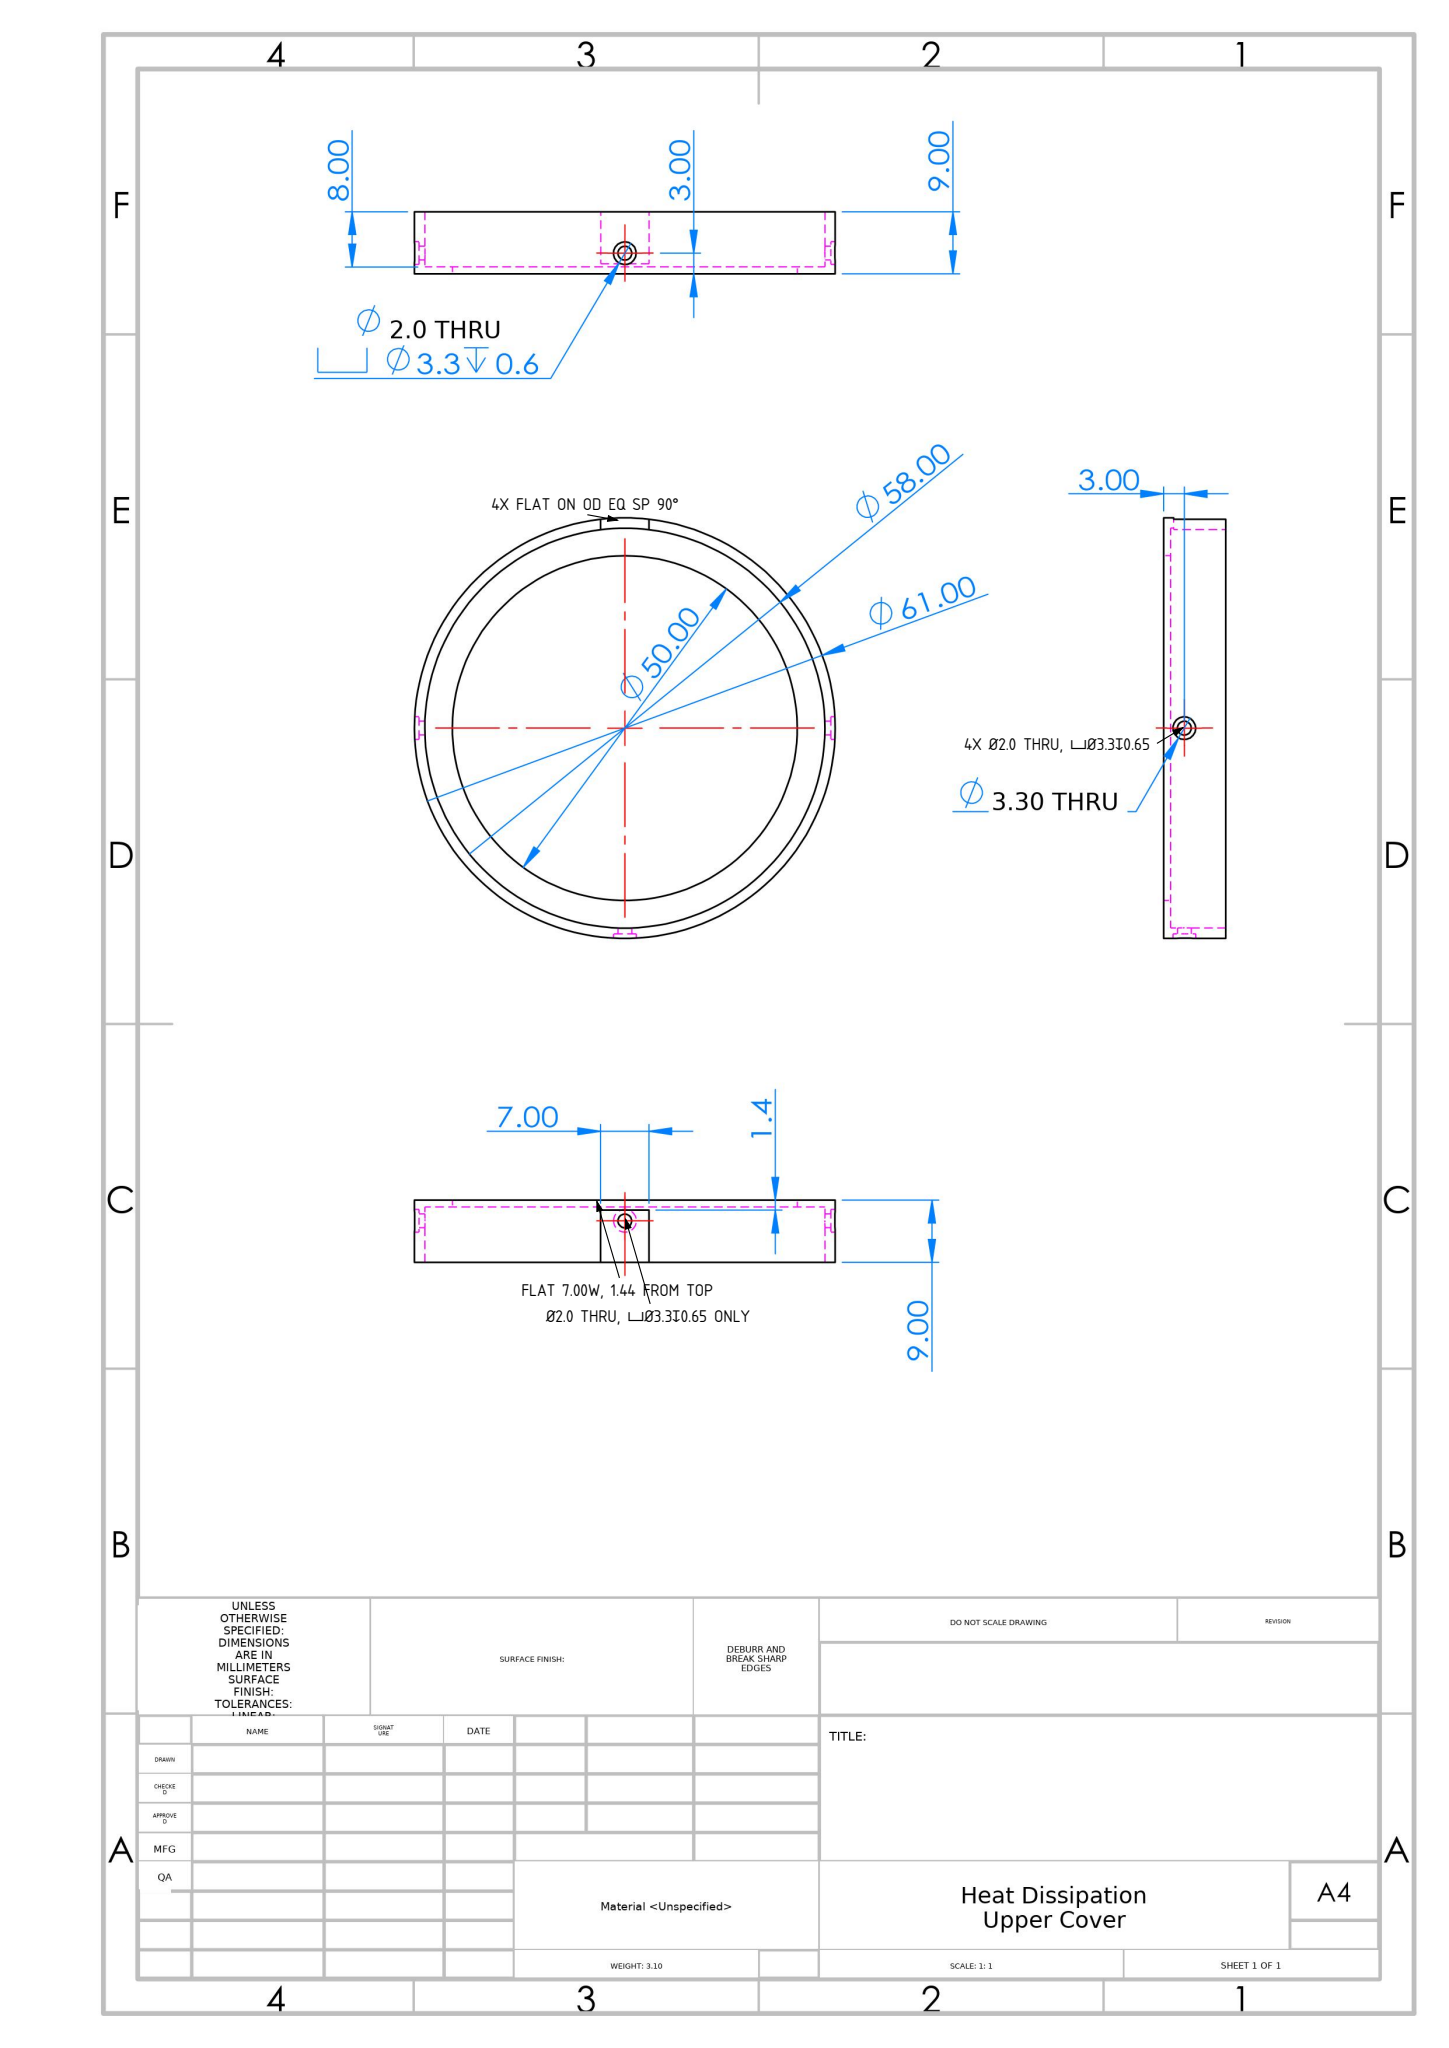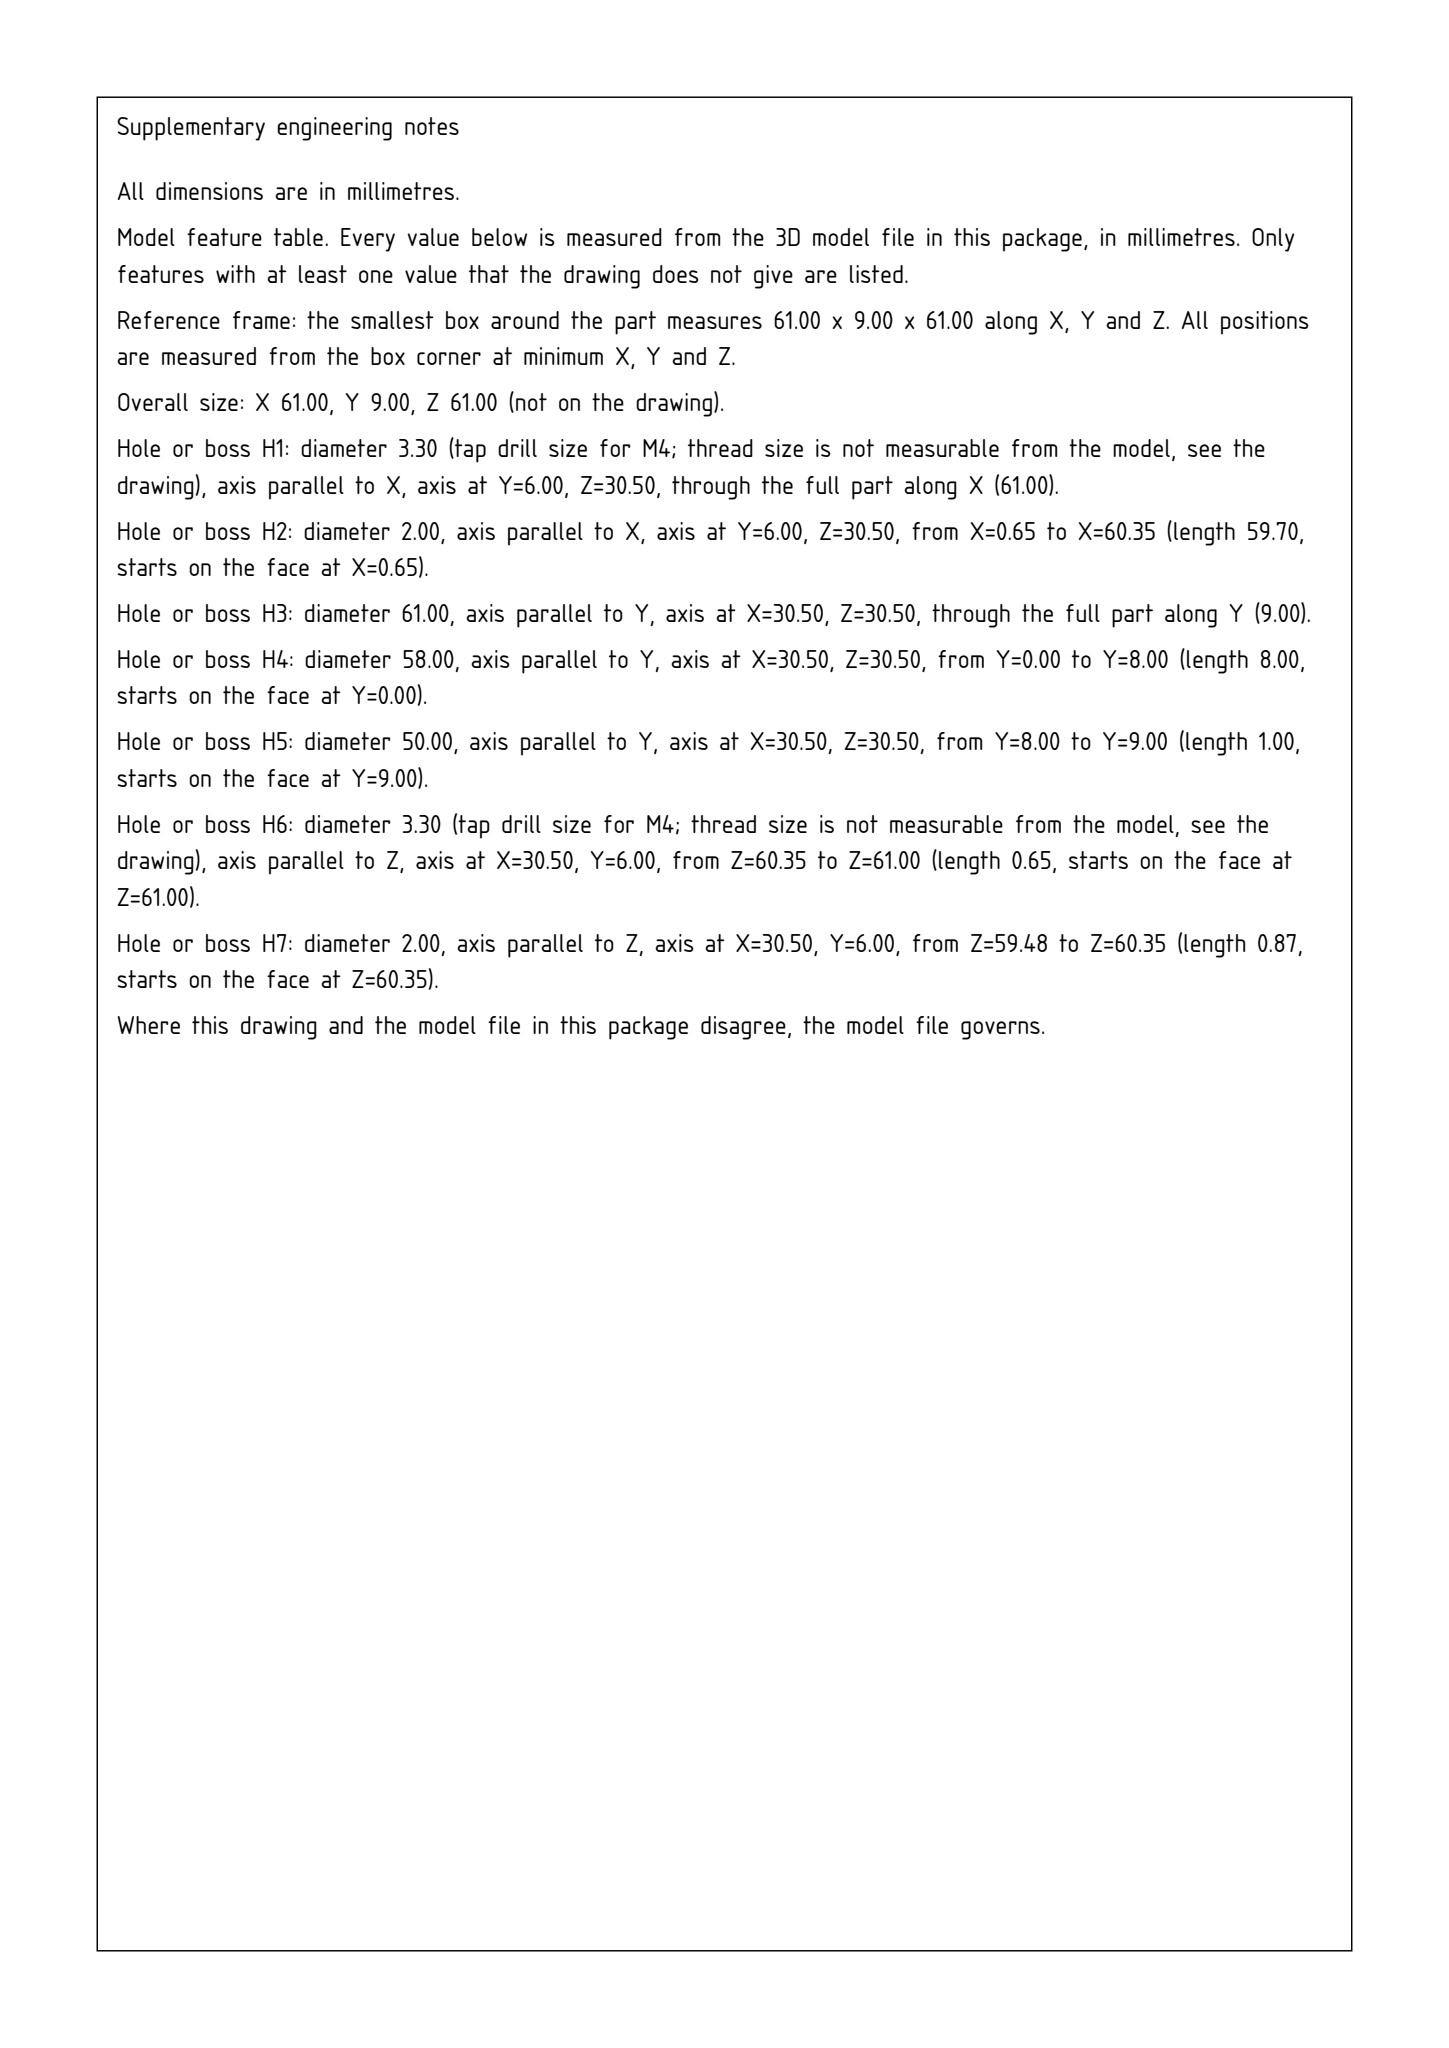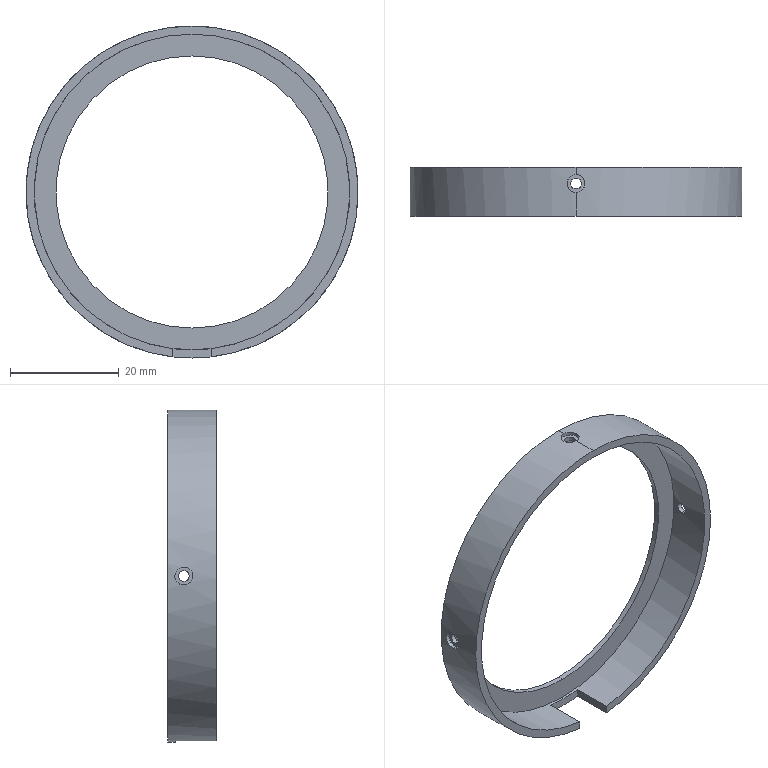Part | SolidWorks | mm | 1 solid | 27 faces | box 61 x 9 x 61 mm | volume 3098 mm3 | cylinder 18 | plane 9 | commonest cylinder face diameters 2 x6 3.3 x6 50 x2 61 x2 58 x2
Drawing notes:
4X Ø2.0 THRU, C'BORE Ø3.3 DP 0.65, EQ SP 90° ON CL | from the solid: Ø2.0 holes: 4 on x-axis + 2 on z-axis faces at y=6, z/x=30.5; Ø3.3 c'bore len 0.65; 4 radial holes 90° apart on X & Z centerlines
4X OD FLAT EQ SP 90°, IN LINE W/ RADIAL HOLES | from the solid: flat planes x=0.65, x=60.35, z=60.35 (and z=0.65) tangent-cut on Ø61 OD, centered on 30.5 i.e. on hole centerlines
OD FLAT 7.00 W x 1.44 AXIAL FROM TOP FACE, 0.65 DEEP RAD | from the solid: side planes x=27.0 & x=34.0 (7.00 wide); y plane 7.56 vs top y=9.0 => 1.44; flat at 60.35 vs R30.5 => 0.65 deep
RADIAL HOLE IS Ø2.0 THRU; Ø3.3 IS C'BORE DP 0.65 ONLY | from the solid: Ø3.3 cyl length 0.65 + Ø2.0 cyl length 0.87 = 1.52 wall (Ø61 to Ø58); Ø3.3 not through
build123d program:
from build123d import *

# Parameters (mm, degrees)
SKETCH2_W          = 7
SKETCH2_H          = 10
CUT_EXTRUDE1_DEPTH = 45.062
CUT_EXTRUDE2_START = 29.85
SKETCH3_R          = 1.65
CUT_EXTRUDE2_DEPTH = 10.65
CIRPATTERN1_COUNT  = 4
SKETCH4_R          = 1
CUT_EXTRUDE3_DEPTH = 45.062
CIRPATTERN3_COUNT  = 4


with BuildPart() as part:
    # Sketch1 → Revolve1 (revolve)
    with BuildSketch(Plane.XY, mode=Mode.PRIVATE) as revolve1_sk:
        Polygon((29, 0), (29, 8), (25, 8), (25, 9), (30.5, 9), (30.5, 0), align=None)
    revolve(revolve1_sk.sketch.rotate(Axis((0, -1.348, 0), (0, 1, 0)), 90), axis=Axis((0, -1.348, 0), (0, 1, 0)))

    # Sketch2 → Cut-Extrude1 (cut, through all)
    with BuildSketch(Plane.XY):
        with Locations((0, 2.56)):
            Rectangle(SKETCH2_W, SKETCH2_H)
    extrude(amount=-CUT_EXTRUDE1_DEPTH, mode=Mode.SUBTRACT)

    # Sketch3 → Cut-Extrude2 (cut)
    with BuildSketch(Plane.XY.offset(CUT_EXTRUDE2_START)):
        with Locations(Location((0, 6, 0), (0, 0, 180))):
            Circle(SKETCH3_R)
    cut_extrude2 = extrude(amount=CUT_EXTRUDE2_DEPTH, mode=Mode.SUBTRACT)

    # CirPattern1: Cut-Extrude2 ×4 about axis, 1 skipped
    cirpattern1_axis = Axis((0, 0, 0), (0, -1, 0))
    add([cut_extrude2.rotate(cirpattern1_axis, i * 360 / CIRPATTERN1_COUNT) for i in range(1, CIRPATTERN1_COUNT) if i not in (2,)], mode=Mode.SUBTRACT)

    # Sketch4 → Cut-Extrude3 (cut, through all)
    with BuildSketch(Plane.XY):
        with Locations(Location((0, 6, 0), (0, 0, 180))):
            Circle(SKETCH4_R)
    cut_extrude3 = extrude(amount=CUT_EXTRUDE3_DEPTH, mode=Mode.SUBTRACT)

    # CirPattern3: Cut-Extrude3 ×4 about axis, 1 skipped
    cirpattern3_axis = Axis((0, -1.348, 0), (0, -1, 0))
    add([cut_extrude3.rotate(cirpattern3_axis, i * 360 / CIRPATTERN3_COUNT) for i in range(1, CIRPATTERN3_COUNT) if i not in (2,)], mode=Mode.SUBTRACT)


solid = part.part